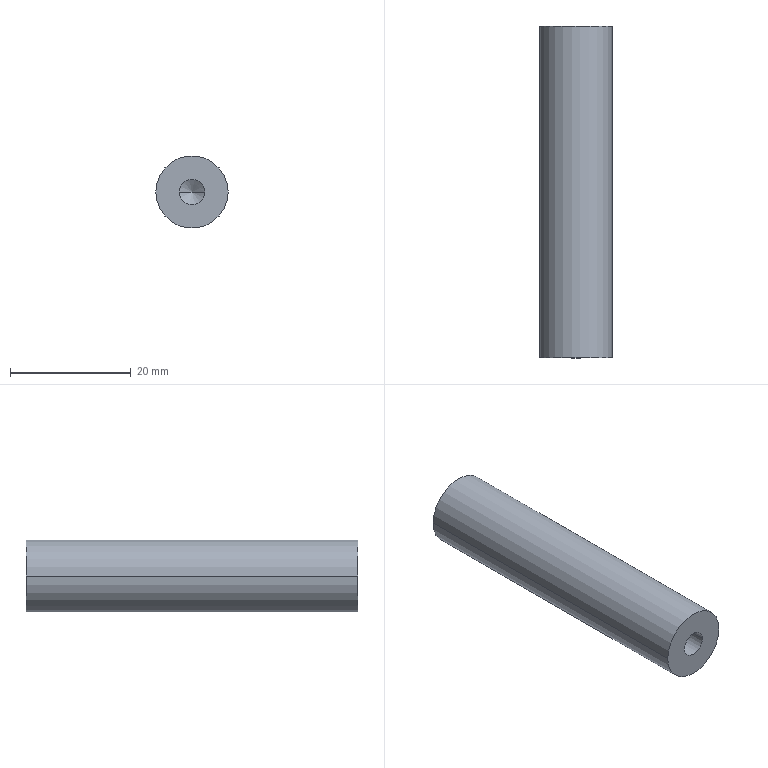Component | SolidWorks | H2020022-0409-1-1 | 1 solid | 12 faces | box 12 x 55 x 12 mm | volume 5865 mm3 | cylinder 6 | cone 4 | plane 2 | commonest cylinder face diameters 4.2 x4 12 x2 | material 45#Steel
build123d program:
from build123d import *

# Parameters (mm, degrees)
SKETCH1_R             = 6
BOSS_EXTRUDE1_DEPTH   = 55
M5_TAPPED_HOLE3_D     = 4.2
M5_TAPPED_HOLE3_DEPTH = 12.4
M5_TAPPED_HOLE3_TIP   = 1.262
M5_TAPPED_HOLE4_D     = 4.2
M5_TAPPED_HOLE4_DEPTH = 12.4
M5_TAPPED_HOLE4_TIP   = 1.262


with BuildPart() as part:
    # Sketch1 → Boss-Extrude1 (new body)
    with BuildSketch(Plane(origin=(0, 0, 0), x_dir=(0, 0, -1), z_dir=(1, 0, 0))):
        Circle(SKETCH1_R)
    extrude(amount=BOSS_EXTRUDE1_DEPTH)

    # M5 Tapped Hole3
    with Locations(Plane(origin=(55, 0, 0), x_dir=(0, 0, -1), z_dir=(1, 0, 0))):
        with Locations((0, 0)):
            Hole(M5_TAPPED_HOLE3_D / 2, depth=M5_TAPPED_HOLE3_DEPTH)
            with Locations((0, 0, -(M5_TAPPED_HOLE3_DEPTH + M5_TAPPED_HOLE3_TIP / 2))):  # 118° drill point
                Cone(0, M5_TAPPED_HOLE3_D / 2, M5_TAPPED_HOLE3_TIP, mode=Mode.SUBTRACT)

    # M5 Tapped Hole4
    with Locations(Plane.ZY):
        with Locations((0, 0)):
            Hole(M5_TAPPED_HOLE4_D / 2, depth=M5_TAPPED_HOLE4_DEPTH)
            with Locations((0, 0, -(M5_TAPPED_HOLE4_DEPTH + M5_TAPPED_HOLE4_TIP / 2))):  # 118° drill point
                Cone(0, M5_TAPPED_HOLE4_D / 2, M5_TAPPED_HOLE4_TIP, mode=Mode.SUBTRACT)


solid = part.part

# Placed as in the assembly
solid = solid.moved(Location((-68.464, 47.013, 307.697), (0, 0, 90)))
STEP:
#1=COLOUR_RGB('',0.7922,0.8196,0.9333);
#2=FILL_AREA_STYLE_COLOUR('',#1);
#3=FILL_AREA_STYLE('',(#2));
#4=SURFACE_STYLE_FILL_AREA(#3);
#5=SURFACE_SIDE_STYLE('',(#4));
#6=SURFACE_STYLE_USAGE(.BOTH.,#5);
#7=PRESENTATION_STYLE_ASSIGNMENT((#6));
#8=CARTESIAN_POINT('',(-2.778,2.339,12.114));
#9=VERTEX_POINT('',#8);
#10=CARTESIAN_POINT('',(-2.613,2.339,12.114));
#11=VERTEX_POINT('',#10);
#12=CARTESIAN_POINT('',(-2.695,2.339,12.114));
#13=DIRECTION('',(0.,-1.,0.));
#14=DIRECTION('',(1.,0.,0.));
#15=AXIS2_PLACEMENT_3D('',#12,#13,#14);
#16=CIRCLE('',#15,0.08268);
#17=EDGE_CURVE('',#9,#11,#16,.T.);
#18=ORIENTED_EDGE('',*,*,#17,.F.);
#19=CARTESIAN_POINT('',(-2.778,1.851,12.114));
#20=VERTEX_POINT('',#19);
#21=CARTESIAN_POINT('',(-2.778,1.851,12.114));
#22=DIRECTION('',(0.,-1.,0.));
#23=VECTOR('',#22,39.37);
#24=LINE('',#21,#23);
#25=EDGE_CURVE('',#9,#20,#24,.T.);
#26=ORIENTED_EDGE('',*,*,#25,.T.);
#27=CARTESIAN_POINT('',(-2.613,1.851,12.114));
#28=VERTEX_POINT('',#27);
#29=CARTESIAN_POINT('',(-2.695,1.851,12.114));
#30=DIRECTION('',(0.,-1.,0.));
#31=DIRECTION('',(1.,0.,0.));
#32=AXIS2_PLACEMENT_3D('',#29,#30,#31);
#33=CIRCLE('',#32,0.08268);
#34=EDGE_CURVE('',#20,#28,#33,.T.);
#35=ORIENTED_EDGE('',*,*,#34,.T.);
#36=CARTESIAN_POINT('',(-2.613,1.851,12.114));
#37=DIRECTION('',(0.,-1.,0.));
#38=VECTOR('',#37,39.37);
#39=LINE('',#36,#38);
#40=EDGE_CURVE('',#11,#28,#39,.T.);
#41=ORIENTED_EDGE('',*,*,#40,.F.);
#42=EDGE_LOOP('',(#18,#26,#35,#41));
#43=FACE_OUTER_BOUND('',#42,.T.);
#44=CARTESIAN_POINT('',(-2.695,1.851,12.114));
#45=DIRECTION('',(0.,-1.,0.));
#46=DIRECTION('',(1.,0.,0.));
#47=AXIS2_PLACEMENT_3D('',#44,#45,#46);
#48=CYLINDRICAL_SURFACE('',#47,0.08268);
#49=ADVANCED_FACE('',(#43),#48,.F.);
#50=CARTESIAN_POINT('',(-2.695,2.389,12.114));
#51=VERTEX_POINT('',#50);
#52=CARTESIAN_POINT('',(-2.613,2.339,12.114));
#53=DIRECTION('',(0.8572,-0.515,0.));
#54=VECTOR('',#53,39.37);
#55=LINE('',#52,#54);
#56=EDGE_CURVE('',#51,#11,#55,.T.);
#57=ORIENTED_EDGE('',*,*,#56,.F.);
#58=CARTESIAN_POINT('',(-2.778,2.339,12.114));
#59=DIRECTION('',(-0.8572,-0.515,-0.));
#60=VECTOR('',#59,39.37);
#61=LINE('',#58,#60);
#62=EDGE_CURVE('',#51,#9,#61,.T.);
#63=ORIENTED_EDGE('',*,*,#62,.T.);
#64=ORIENTED_EDGE('',*,*,#17,.T.);
#65=EDGE_LOOP('',(#57,#63,#64));
#66=FACE_OUTER_BOUND('',#65,.T.);
#67=CARTESIAN_POINT('',(-2.695,2.339,12.114));
#68=DIRECTION('',(0.,-1.,0.));
#69=DIRECTION('',(1.,0.,0.));
#70=AXIS2_PLACEMENT_3D('',#67,#68,#69);
#71=CONICAL_SURFACE('',#70,0.08268,1.03);
#72=ADVANCED_FACE('',(#66),#71,.F.);
#73=CARTESIAN_POINT('',(-2.613,3.528,12.114));
#74=VERTEX_POINT('',#73);
#75=CARTESIAN_POINT('',(-2.778,3.528,12.114));
#76=VERTEX_POINT('',#75);
#77=CARTESIAN_POINT('',(-2.695,3.528,12.114));
#78=DIRECTION('',(0.,1.,0.));
#79=DIRECTION('',(-1.,0.,0.));
#80=AXIS2_PLACEMENT_3D('',#77,#78,#79);
#81=CIRCLE('',#80,0.08268);
#82=EDGE_CURVE('',#74,#76,#81,.T.);
#83=ORIENTED_EDGE('',*,*,#82,.F.);
#84=CARTESIAN_POINT('',(-2.613,4.016,12.114));
#85=VERTEX_POINT('',#84);
#86=CARTESIAN_POINT('',(-2.613,4.016,12.114));
#87=DIRECTION('',(0.,1.,0.));
#88=VECTOR('',#87,39.37);
#89=LINE('',#86,#88);
#90=EDGE_CURVE('',#74,#85,#89,.T.);
#91=ORIENTED_EDGE('',*,*,#90,.T.);
#92=CARTESIAN_POINT('',(-2.778,4.016,12.114));
#93=VERTEX_POINT('',#92);
#94=CARTESIAN_POINT('',(-2.695,4.016,12.114));
#95=DIRECTION('',(0.,1.,0.));
#96=DIRECTION('',(-1.,0.,0.));
#97=AXIS2_PLACEMENT_3D('',#94,#95,#96);
#98=CIRCLE('',#97,0.08268);
#99=EDGE_CURVE('',#85,#93,#98,.T.);
#100=ORIENTED_EDGE('',*,*,#99,.T.);
#101=CARTESIAN_POINT('',(-2.778,4.016,12.114));
#102=DIRECTION('',(0.,1.,0.));
#103=VECTOR('',#102,39.37);
#104=LINE('',#101,#103);
#105=EDGE_CURVE('',#76,#93,#104,.T.);
#106=ORIENTED_EDGE('',*,*,#105,.F.);
#107=EDGE_LOOP('',(#83,#91,#100,#106));
#108=FACE_OUTER_BOUND('',#107,.T.);
#109=CARTESIAN_POINT('',(-2.695,4.016,12.114));
#110=DIRECTION('',(0.,1.,0.));
#111=DIRECTION('',(-1.,0.,0.));
#112=AXIS2_PLACEMENT_3D('',#109,#110,#111);
#113=CYLINDRICAL_SURFACE('',#112,0.08268);
#114=ADVANCED_FACE('',(#108),#113,.F.);
#115=CARTESIAN_POINT('',(-2.695,3.478,12.114));
#116=VERTEX_POINT('',#115);
#117=CARTESIAN_POINT('',(-2.778,3.528,12.114));
#118=DIRECTION('',(-0.8572,0.515,-0.));
#119=VECTOR('',#118,39.37);
#120=LINE('',#117,#119);
#121=EDGE_CURVE('',#116,#76,#120,.T.);
#122=ORIENTED_EDGE('',*,*,#121,.F.);
#123=CARTESIAN_POINT('',(-2.613,3.528,12.114));
#124=DIRECTION('',(0.8572,0.515,0.));
#125=VECTOR('',#124,39.37);
#126=LINE('',#123,#125);
#127=EDGE_CURVE('',#116,#74,#126,.T.);
#128=ORIENTED_EDGE('',*,*,#127,.T.);
#129=ORIENTED_EDGE('',*,*,#82,.T.);
#130=EDGE_LOOP('',(#122,#128,#129));
#131=FACE_OUTER_BOUND('',#130,.T.);
#132=CARTESIAN_POINT('',(-2.695,3.528,12.114));
#133=DIRECTION('',(0.,1.,0.));
#134=DIRECTION('',(-1.,0.,0.));
#135=AXIS2_PLACEMENT_3D('',#132,#133,#134);
#136=CONICAL_SURFACE('',#135,0.08268,1.03);
#137=ADVANCED_FACE('',(#131),#136,.F.);
#138=CARTESIAN_POINT('',(-2.932,4.016,12.114));
#139=VERTEX_POINT('',#138);
#140=CARTESIAN_POINT('',(-2.459,4.016,12.114));
#141=VERTEX_POINT('',#140);
#142=CARTESIAN_POINT('',(-2.695,4.016,12.114));
#143=DIRECTION('',(0.,1.,0.));
#144=DIRECTION('',(-1.,0.,0.));
#145=AXIS2_PLACEMENT_3D('',#142,#143,#144);
#146=CIRCLE('',#145,0.2362);
#147=EDGE_CURVE('',#139,#141,#146,.T.);
#148=ORIENTED_EDGE('',*,*,#147,.F.);
#149=CARTESIAN_POINT('',(-2.932,1.851,12.114));
#150=VERTEX_POINT('',#149);
#151=CARTESIAN_POINT('',(-2.932,4.016,12.114));
#152=DIRECTION('',(0.,-1.,0.));
#153=VECTOR('',#152,39.37);
#154=LINE('',#151,#153);
#155=EDGE_CURVE('',#139,#150,#154,.T.);
#156=ORIENTED_EDGE('',*,*,#155,.T.);
#157=CARTESIAN_POINT('',(-2.459,1.851,12.114));
#158=VERTEX_POINT('',#157);
#159=CARTESIAN_POINT('',(-2.695,1.851,12.114));
#160=DIRECTION('',(0.,1.,0.));
#161=DIRECTION('',(-1.,0.,0.));
#162=AXIS2_PLACEMENT_3D('',#159,#160,#161);
#163=CIRCLE('',#162,0.2362);
#164=EDGE_CURVE('',#150,#158,#163,.T.);
#165=ORIENTED_EDGE('',*,*,#164,.T.);
#166=CARTESIAN_POINT('',(-2.459,4.016,12.114));
#167=DIRECTION('',(0.,-1.,0.));
#168=VECTOR('',#167,39.37);
#169=LINE('',#166,#168);
#170=EDGE_CURVE('',#141,#158,#169,.T.);
#171=ORIENTED_EDGE('',*,*,#170,.F.);
#172=EDGE_LOOP('',(#148,#156,#165,#171));
#173=FACE_OUTER_BOUND('',#172,.T.);
#174=CARTESIAN_POINT('',(-2.695,4.016,12.114));
#175=DIRECTION('',(0.,-1.,0.));
#176=DIRECTION('',(1.,0.,0.));
#177=AXIS2_PLACEMENT_3D('',#174,#175,#176);
#178=CYLINDRICAL_SURFACE('',#177,0.2362);
#179=ADVANCED_FACE('',(#173),#178,.T.);
#180=ORIENTED_EDGE('',*,*,#155,.F.);
#181=CARTESIAN_POINT('',(-2.695,4.016,12.114));
#182=DIRECTION('',(0.,1.,0.));
#183=DIRECTION('',(-1.,0.,0.));
#184=AXIS2_PLACEMENT_3D('',#181,#182,#183);
#185=CIRCLE('',#184,0.2362);
#186=EDGE_CURVE('',#141,#139,#185,.T.);
#187=ORIENTED_EDGE('',*,*,#186,.F.);
#188=ORIENTED_EDGE('',*,*,#170,.T.);
#189=CARTESIAN_POINT('',(-2.695,1.851,12.114));
#190=DIRECTION('',(0.,1.,0.));
#191=DIRECTION('',(-1.,0.,0.));
#192=AXIS2_PLACEMENT_3D('',#189,#190,#191);
#193=CIRCLE('',#192,0.2362);
#194=EDGE_CURVE('',#158,#150,#193,.T.);
#195=ORIENTED_EDGE('',*,*,#194,.T.);
#196=EDGE_LOOP('',(#180,#187,#188,#195));
#197=FACE_OUTER_BOUND('',#196,.T.);
#198=CARTESIAN_POINT('',(-2.695,4.016,12.114));
#199=DIRECTION('',(0.,-1.,0.));
#200=DIRECTION('',(1.,0.,0.));
#201=AXIS2_PLACEMENT_3D('',#198,#199,#200);
#202=CYLINDRICAL_SURFACE('',#201,0.2362);
#203=ADVANCED_FACE('',(#197),#202,.T.);
#204=CARTESIAN_POINT('',(-2.695,4.016,12.114));
#205=DIRECTION('',(0.,1.,0.));
#206=DIRECTION('',(-1.,0.,0.));
#207=AXIS2_PLACEMENT_3D('',#204,#205,#206);
#208=CIRCLE('',#207,0.08268);
#209=EDGE_CURVE('',#93,#85,#208,.T.);
#210=ORIENTED_EDGE('',*,*,#209,.F.);
#211=ORIENTED_EDGE('',*,*,#99,.F.);
#212=EDGE_LOOP('',(#210,#211));
#213=FACE_BOUND('',#212,.T.);
#214=ORIENTED_EDGE('',*,*,#186,.T.);
#215=ORIENTED_EDGE('',*,*,#147,.T.);
#216=EDGE_LOOP('',(#214,#215));
#217=FACE_OUTER_BOUND('',#216,.T.);
#218=CARTESIAN_POINT('',(-2.695,4.016,12.114));
#219=DIRECTION('',(0.,1.,0.));
#220=DIRECTION('',(-1.,0.,-0.));
#221=AXIS2_PLACEMENT_3D('',#218,#219,#220);
#222=PLANE('',#221);
#223=ADVANCED_FACE('',(#213,#217),#222,.T.);
#224=CARTESIAN_POINT('',(-2.695,1.851,12.114));
#225=DIRECTION('',(0.,-1.,0.));
#226=DIRECTION('',(1.,0.,0.));
#227=AXIS2_PLACEMENT_3D('',#224,#225,#226);
#228=CIRCLE('',#227,0.08268);
#229=EDGE_CURVE('',#28,#20,#228,.T.);
#230=ORIENTED_EDGE('',*,*,#229,.F.);
#231=ORIENTED_EDGE('',*,*,#34,.F.);
#232=EDGE_LOOP('',(#230,#231));
#233=FACE_BOUND('',#232,.T.);
#234=ORIENTED_EDGE('',*,*,#194,.F.);
#235=ORIENTED_EDGE('',*,*,#164,.F.);
#236=EDGE_LOOP('',(#234,#235));
#237=FACE_OUTER_BOUND('',#236,.T.);
#238=CARTESIAN_POINT('',(-2.695,1.851,12.114));
#239=DIRECTION('',(0.,1.,0.));
#240=DIRECTION('',(-1.,0.,-0.));
#241=AXIS2_PLACEMENT_3D('',#238,#239,#240);
#242=PLANE('',#241);
#243=ADVANCED_FACE('',(#233,#237),#242,.F.);
#244=ORIENTED_EDGE('',*,*,#127,.F.);
#245=ORIENTED_EDGE('',*,*,#121,.T.);
#246=CARTESIAN_POINT('',(-2.695,3.528,12.114));
#247=DIRECTION('',(0.,1.,0.));
#248=DIRECTION('',(-1.,0.,0.));
#249=AXIS2_PLACEMENT_3D('',#246,#247,#248);
#250=CIRCLE('',#249,0.08268);
#251=EDGE_CURVE('',#76,#74,#250,.T.);
#252=ORIENTED_EDGE('',*,*,#251,.T.);
#253=EDGE_LOOP('',(#244,#245,#252));
#254=FACE_OUTER_BOUND('',#253,.T.);
#255=CARTESIAN_POINT('',(-2.695,3.528,12.114));
#256=DIRECTION('',(0.,1.,0.));
#257=DIRECTION('',(-1.,0.,0.));
#258=AXIS2_PLACEMENT_3D('',#255,#256,#257);
#259=CONICAL_SURFACE('',#258,0.08268,1.03);
#260=ADVANCED_FACE('',(#254),#259,.F.);
#261=ORIENTED_EDGE('',*,*,#90,.F.);
#262=ORIENTED_EDGE('',*,*,#251,.F.);
#263=ORIENTED_EDGE('',*,*,#105,.T.);
#264=ORIENTED_EDGE('',*,*,#209,.T.);
#265=EDGE_LOOP('',(#261,#262,#263,#264));
#266=FACE_OUTER_BOUND('',#265,.T.);
#267=CARTESIAN_POINT('',(-2.695,4.016,12.114));
#268=DIRECTION('',(0.,1.,0.));
#269=DIRECTION('',(-1.,0.,0.));
#270=AXIS2_PLACEMENT_3D('',#267,#268,#269);
#271=CYLINDRICAL_SURFACE('',#270,0.08268);
#272=ADVANCED_FACE('',(#266),#271,.F.);
#273=ORIENTED_EDGE('',*,*,#62,.F.);
#274=ORIENTED_EDGE('',*,*,#56,.T.);
#275=CARTESIAN_POINT('',(-2.695,2.339,12.114));
#276=DIRECTION('',(0.,-1.,0.));
#277=DIRECTION('',(1.,0.,0.));
#278=AXIS2_PLACEMENT_3D('',#275,#276,#277);
#279=CIRCLE('',#278,0.08268);
#280=EDGE_CURVE('',#11,#9,#279,.T.);
#281=ORIENTED_EDGE('',*,*,#280,.T.);
#282=EDGE_LOOP('',(#273,#274,#281));
#283=FACE_OUTER_BOUND('',#282,.T.);
#284=CARTESIAN_POINT('',(-2.695,2.339,12.114));
#285=DIRECTION('',(0.,-1.,0.));
#286=DIRECTION('',(1.,0.,0.));
#287=AXIS2_PLACEMENT_3D('',#284,#285,#286);
#288=CONICAL_SURFACE('',#287,0.08268,1.03);
#289=ADVANCED_FACE('',(#283),#288,.F.);
#290=ORIENTED_EDGE('',*,*,#25,.F.);
#291=ORIENTED_EDGE('',*,*,#280,.F.);
#292=ORIENTED_EDGE('',*,*,#40,.T.);
#293=ORIENTED_EDGE('',*,*,#229,.T.);
#294=EDGE_LOOP('',(#290,#291,#292,#293));
#295=FACE_OUTER_BOUND('',#294,.T.);
#296=CARTESIAN_POINT('',(-2.695,1.851,12.114));
#297=DIRECTION('',(0.,-1.,0.));
#298=DIRECTION('',(1.,0.,0.));
#299=AXIS2_PLACEMENT_3D('',#296,#297,#298);
#300=CYLINDRICAL_SURFACE('',#299,0.08268);
#301=ADVANCED_FACE('',(#295),#300,.F.);
#302=CLOSED_SHELL('',(#49,#72,#114,#137,#179,#203,#223,#243,#260,#272,#289,#301));
#303=MANIFOLD_SOLID_BREP('',#302);
#304=STYLED_ITEM('',(#7),#303);
#305=(LENGTH_UNIT()NAMED_UNIT(*)SI_UNIT($,.METRE.));
#306=LENGTH_MEASURE_WITH_UNIT(LENGTH_MEASURE(0.0254),#305);
#307=DIMENSIONAL_EXPONENTS(1.,0.,0.,0.,0.,0.,0.);
#308=(CONVERSION_BASED_UNIT('',#306)LENGTH_UNIT()NAMED_UNIT(#307));
#309=UNCERTAINTY_MEASURE_WITH_UNIT(LENGTH_MEASURE(0.00001),#308,'','');
#310=(NAMED_UNIT(*)PLANE_ANGLE_UNIT()SI_UNIT($,.RADIAN.));
#311=(NAMED_UNIT(*)SI_UNIT($,.STERADIAN.)SOLID_ANGLE_UNIT());
#312=(GEOMETRIC_REPRESENTATION_CONTEXT(3)GLOBAL_UNCERTAINTY_ASSIGNED_CONTEXT((#309))GLOBAL_UNIT_ASSIGNED_CONTEXT((#308,#310,#311))REPRESENTATION_CONTEXT('',''));
#313=MECHANICAL_DESIGN_GEOMETRIC_PRESENTATION_REPRESENTATION('',(#304),#312);
#314=PRESENTATION_LAYER_ASSIGNMENT('','',(#304));
#315=CARTESIAN_POINT('',(0.,0.,0.));
#316=DIRECTION('',(0.,0.,1.));
#317=DIRECTION('',(1.,0.,0.));
#318=AXIS2_PLACEMENT_3D('',#315,#316,#317);
#319=(LENGTH_UNIT()NAMED_UNIT(*)SI_UNIT($,.METRE.));
#320=LENGTH_MEASURE_WITH_UNIT(LENGTH_MEASURE(0.0254),#319);
#321=DIMENSIONAL_EXPONENTS(1.,0.,0.,0.,0.,0.,0.);
#322=(CONVERSION_BASED_UNIT('',#320)LENGTH_UNIT()NAMED_UNIT(#321));
#323=UNCERTAINTY_MEASURE_WITH_UNIT(LENGTH_MEASURE(0.00001),#322,'','');
#324=(NAMED_UNIT(*)PLANE_ANGLE_UNIT()SI_UNIT($,.RADIAN.));
#325=(NAMED_UNIT(*)SI_UNIT($,.STERADIAN.)SOLID_ANGLE_UNIT());
#326=(GEOMETRIC_REPRESENTATION_CONTEXT(3)GLOBAL_UNCERTAINTY_ASSIGNED_CONTEXT((#323))GLOBAL_UNIT_ASSIGNED_CONTEXT((#322,#324,#325))REPRESENTATION_CONTEXT('',''));
#327=ADVANCED_BREP_SHAPE_REPRESENTATION('',(#303,#318),#326);